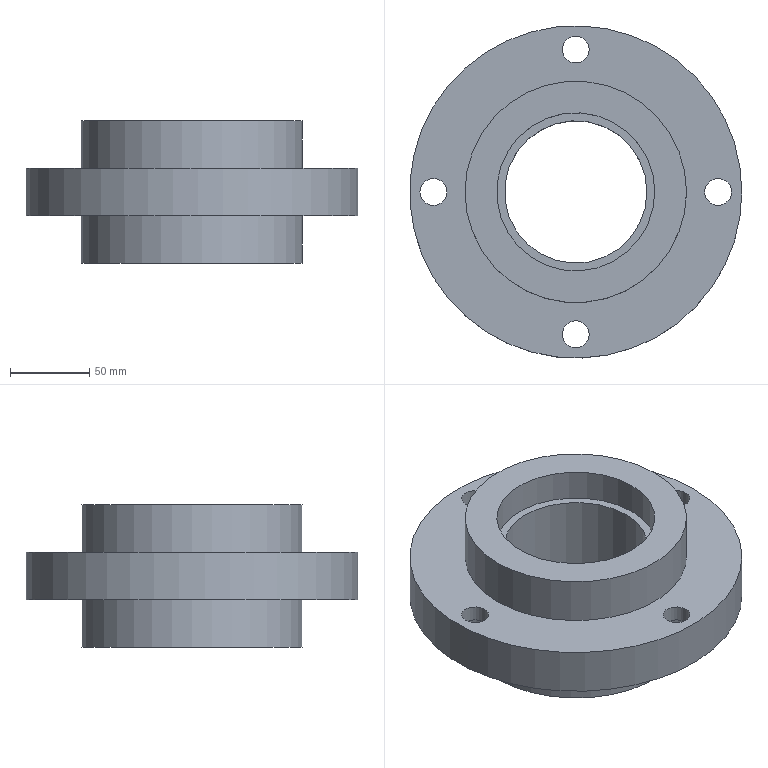Component | NX | FLANGE | 1 solid | 22 faces | volume 1308756 mm3 | cylinder 13 | plane 9 | commonest cylinder face diameters 17 x4 26 x4 140 x2 90 x1 210 x1 100 x1